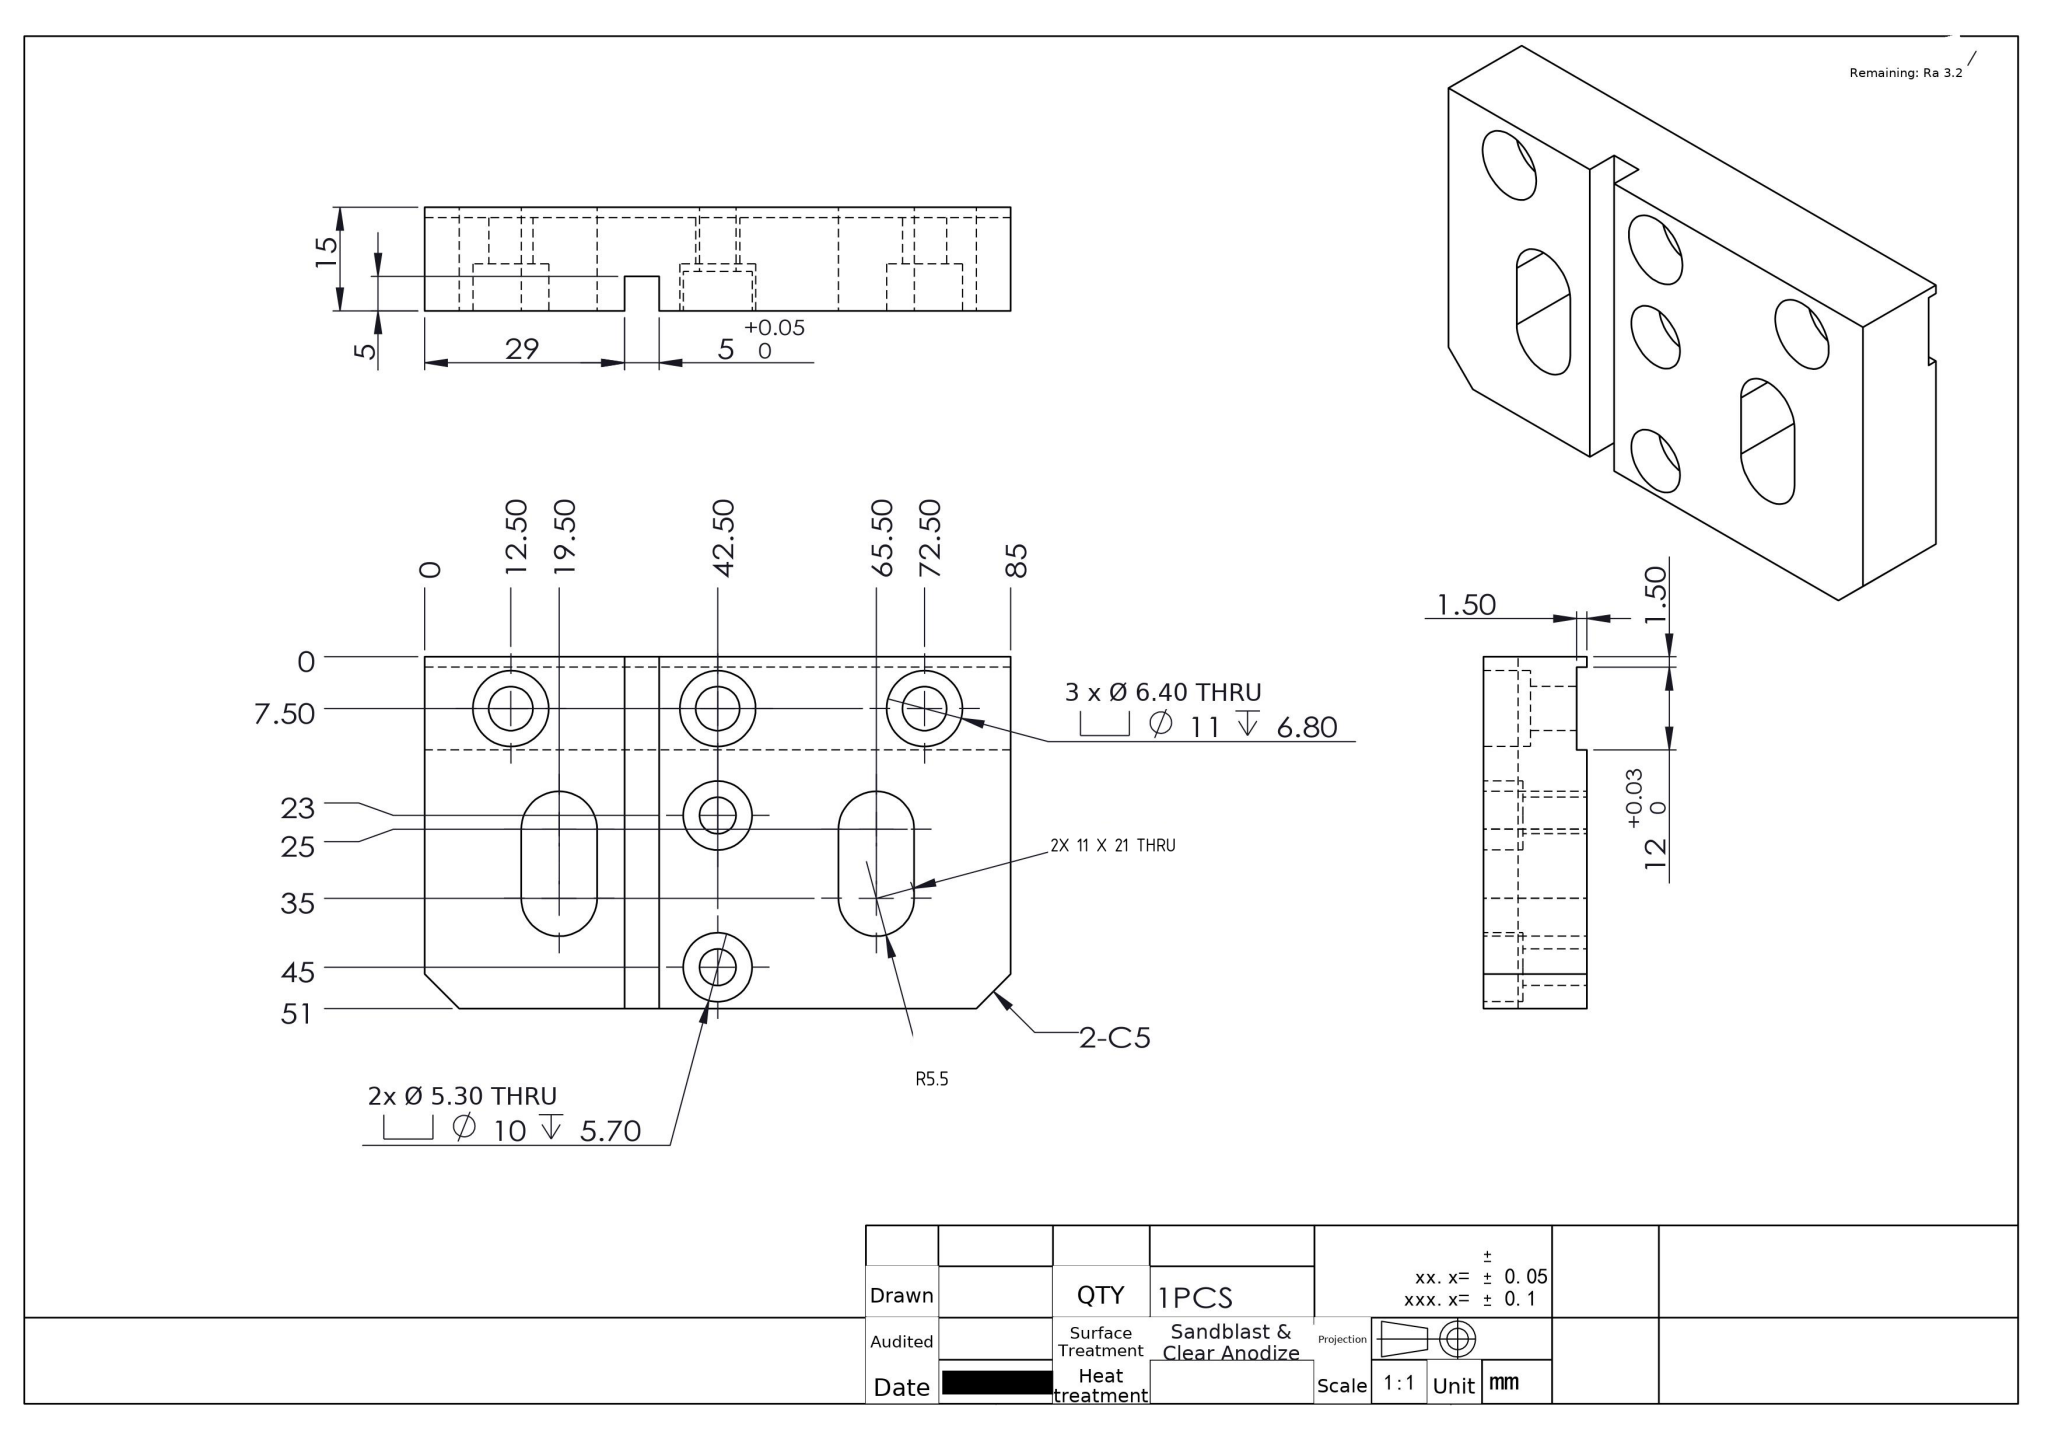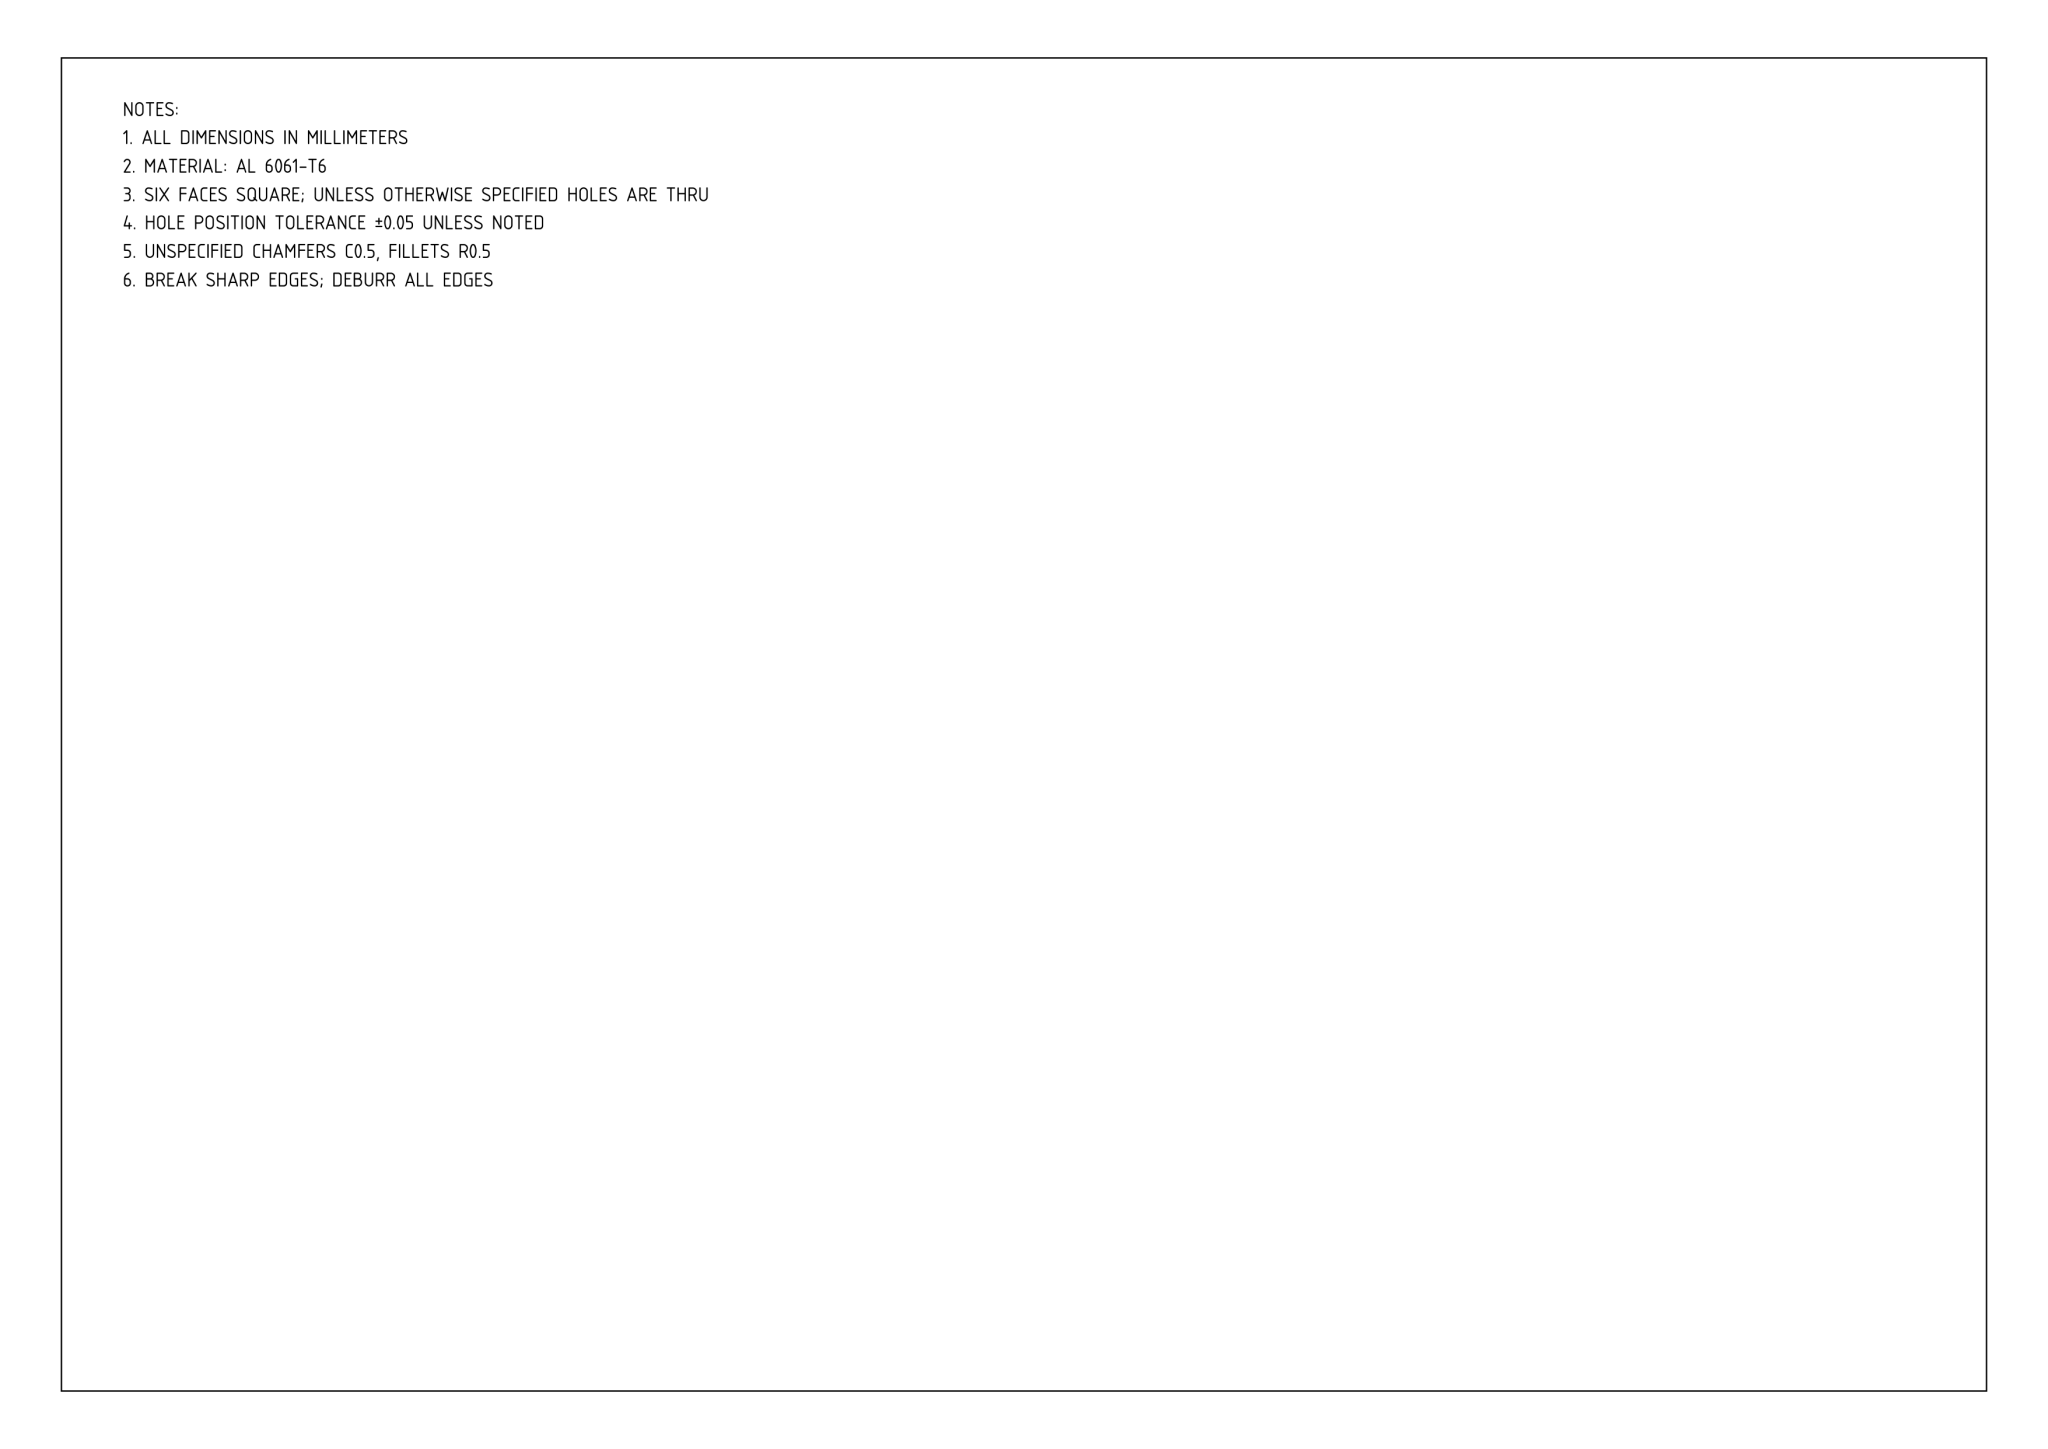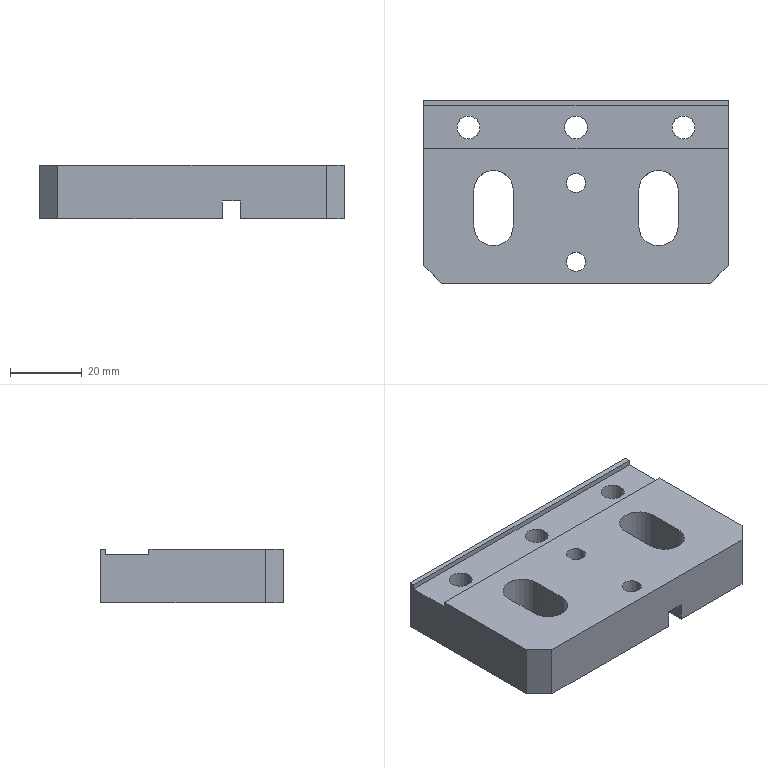Part | NX | mm | 1 solid | 49 faces | box 85 x 51 x 15 mm | volume 51803 mm3 | plane 25 | cylinder 24 | commonest cylinder face diameters 11 x10 6.4 x6 10 x4 5.3 x4